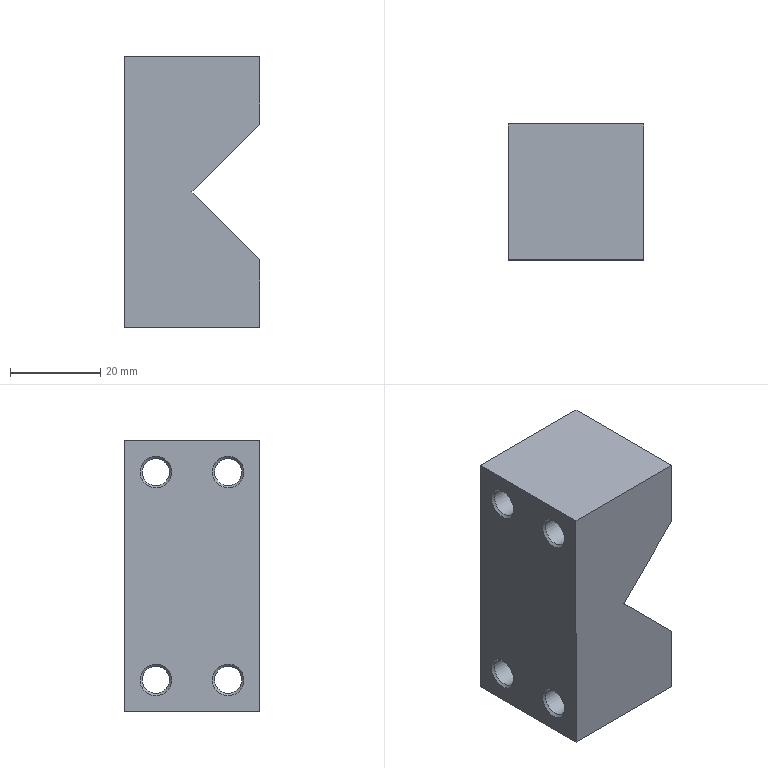Component | NX | V_BLOCK | 1 solid | 21 faces | volume 43837 mm3 | plane 9 | cone 8 | cylinder 4 | commonest cylinder face diameters 6 x4